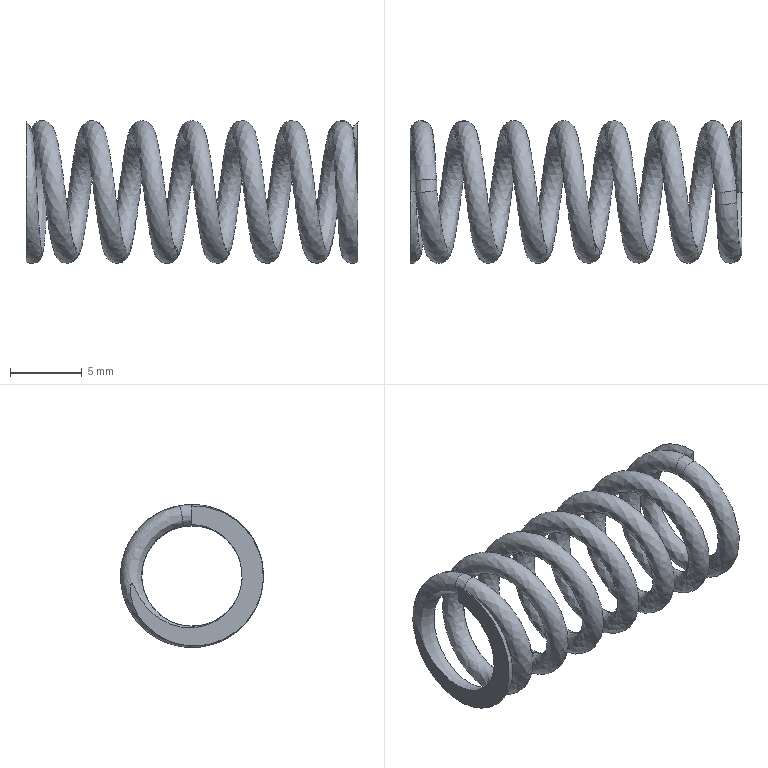Component | NX | SPRING | 1 solid | 9 faces | volume 351 mm3 | spline 5 | plane 4